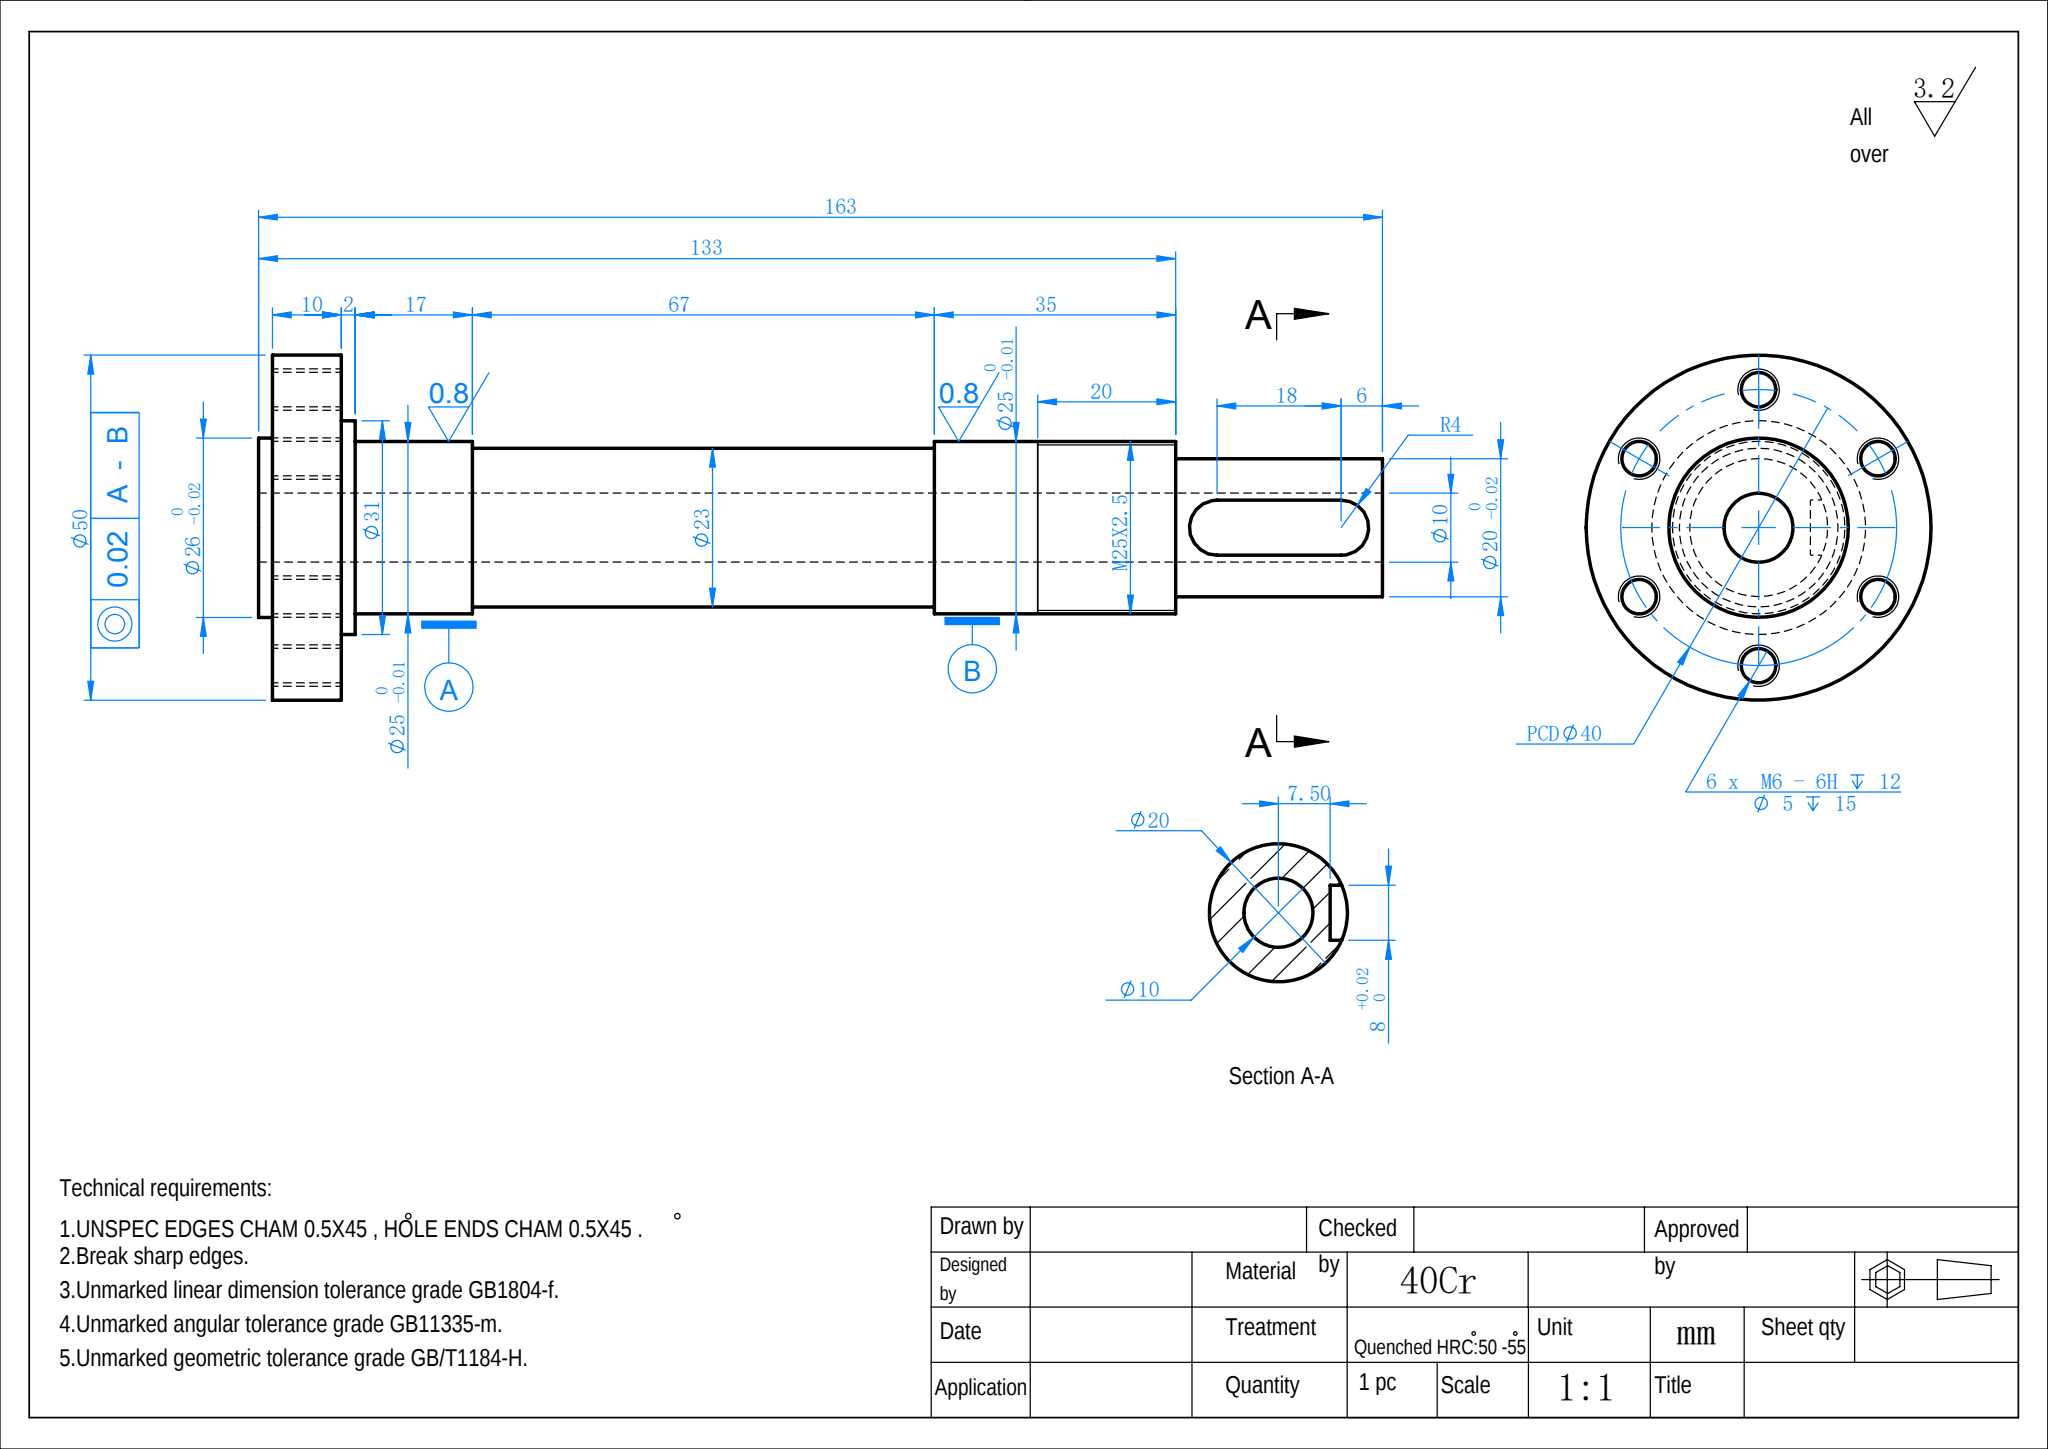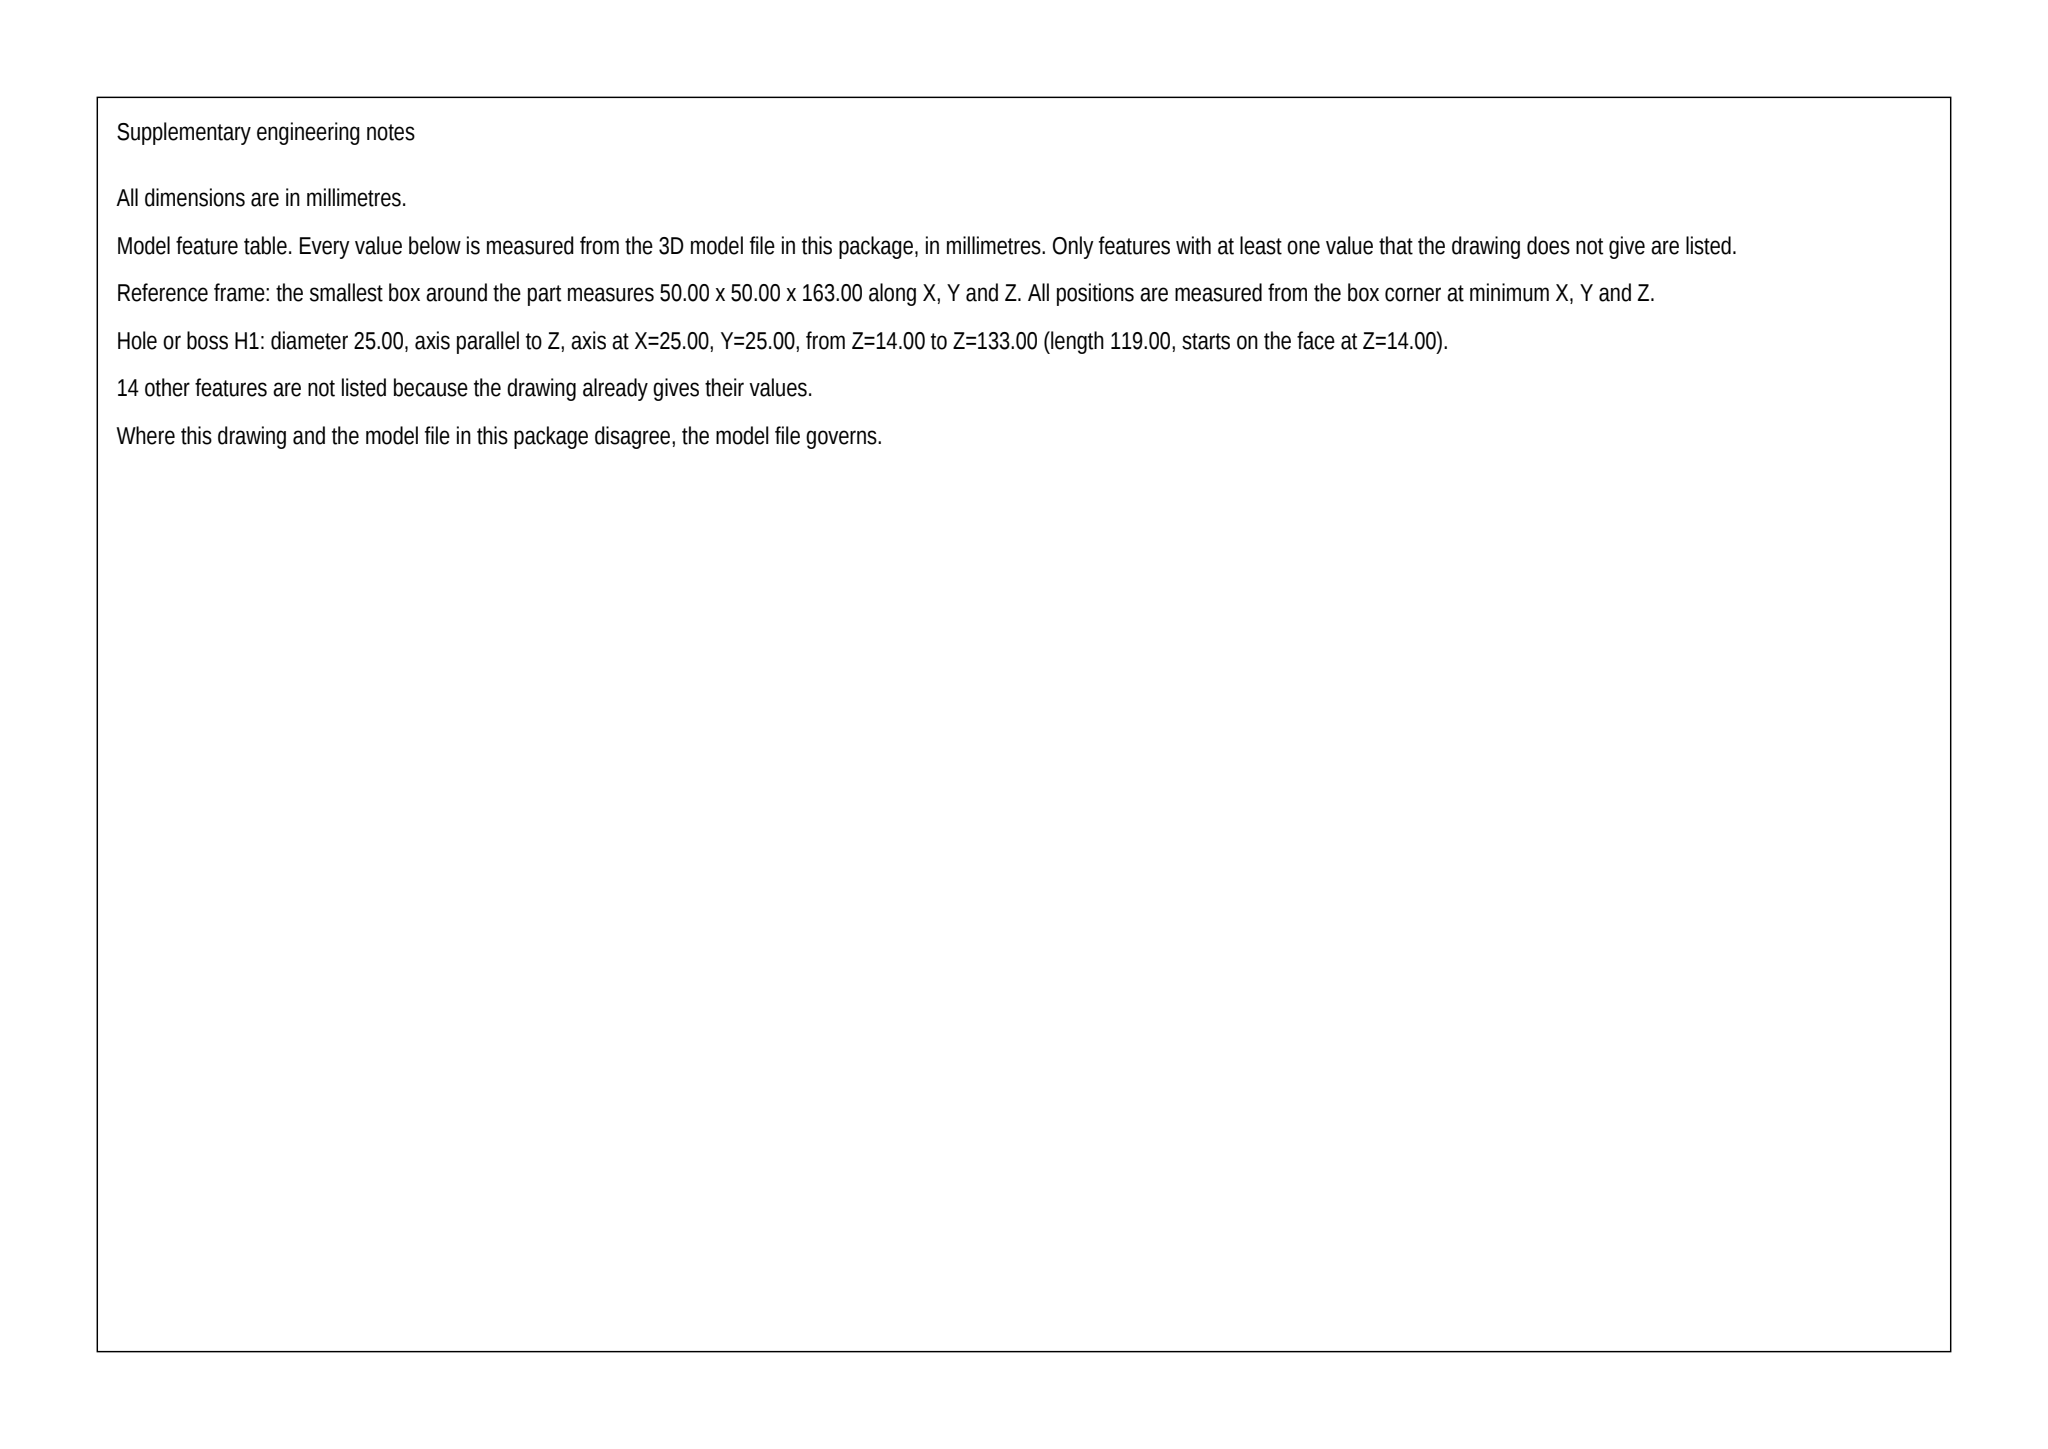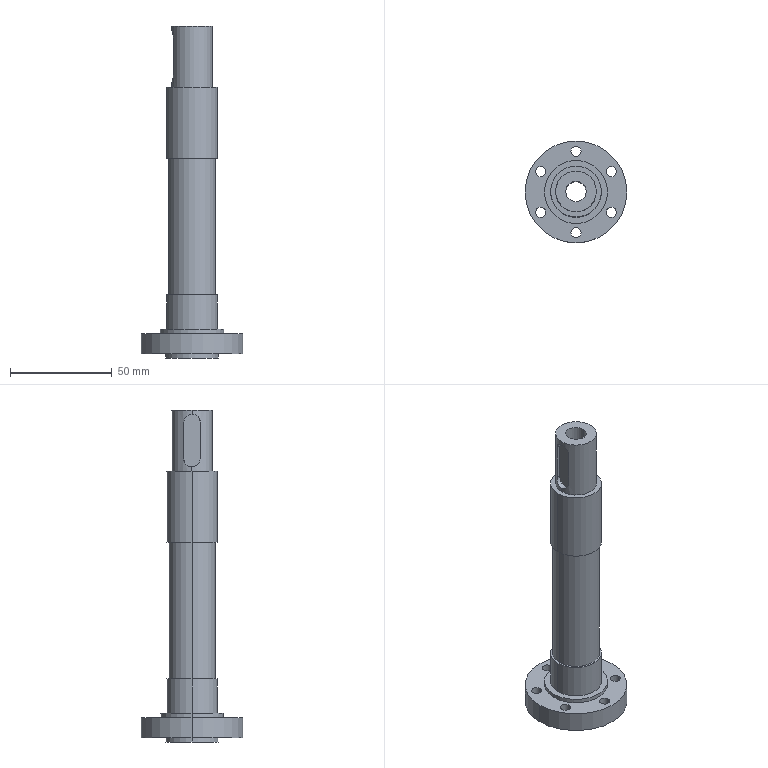Part | SolidWorks | mm | 1 solid | 42 faces | box 50 x 50 x 163 mm | volume 70577 mm3 | cylinder 31 | plane 11 | commonest cylinder face diameters 5 x12 25 x4 8 x3 10 x2 20 x2 23 x2 31 x2 26 x2
build123d program:
from build123d import *

# Parameters (mm, degrees)
SKETCH1_R           = 25
BOSS_EXTRUDE1_DEPTH = 10
SKETCH2_R           = 13
BOSS_EXTRUDE2_DEPTH = 2
SKETCH3_R           = 15.5
BOSS_EXTRUDE3_DEPTH = 2
SKETCH4_R           = 12.5
BOSS_EXTRUDE4_DEPTH = 17
SKETCH5_R           = 11.5
BOSS_EXTRUDE5_DEPTH = 67
SKETCH6_R           = 12.5
BOSS_EXTRUDE6_DEPTH = 35
SKETCH7_R           = 10
BOSS_EXTRUDE7_DEPTH = 30
CIRPATTERN1_COUNT   = 6
SKETCH11_R          = 5
CUT_EXTRUDE1_DEPTH  = 167.79
CUT_EXTRUDE2_DEPTH  = 2.5


with BuildPart() as part:
    # Sketch1 → Boss-Extrude1 (new body)
    with BuildSketch(Plane.XY):
        Circle(SKETCH1_R)
    extrude(amount=BOSS_EXTRUDE1_DEPTH)

    # Sketch2 → Boss-Extrude2 (add)
    with BuildSketch(Plane(origin=(0, 0, 0), x_dir=(-1, 0, 0), z_dir=(0, 0, -1))):
        with Locations(Location((0, 0, 0), (0, 0, 180))):
            Circle(SKETCH2_R)
    extrude(amount=BOSS_EXTRUDE2_DEPTH)

    # Sketch3 → Boss-Extrude3 (add)
    with BuildSketch(Plane.XY.offset(10)):
        Circle(SKETCH3_R)
    extrude(amount=BOSS_EXTRUDE3_DEPTH)

    # Sketch4 → Boss-Extrude4 (add)
    with BuildSketch(Plane.XY.offset(12)):
        Circle(SKETCH4_R)
    extrude(amount=BOSS_EXTRUDE4_DEPTH)

    # Sketch5 → Boss-Extrude5 (add)
    with BuildSketch(Plane.XY.offset(29)):
        Circle(SKETCH5_R)
    extrude(amount=BOSS_EXTRUDE5_DEPTH)

    # Sketch6 → Boss-Extrude6 (add)
    with BuildSketch(Plane.XY.offset(96)):
        Circle(SKETCH6_R)
    extrude(amount=BOSS_EXTRUDE6_DEPTH)

    # Sketch7 → Boss-Extrude7 (add)
    with BuildSketch(Plane.XY.offset(131)):
        Circle(SKETCH7_R)
    extrude(amount=BOSS_EXTRUDE7_DEPTH)

    # Sketch10 → M6 Tapped Hole1 (revolve, cut)
    with BuildSketch(Plane(origin=(0, 20, 0), x_dir=(0, 1, 0), z_dir=(1, 0, 0))):
        Polygon((0, 0), (0, 16.502), (2.5, 15), (2.5, 0), align=None)
    m6_tapped_hole1 = revolve(axis=Axis((0, 20, -6.35), (0, 0, 1)), mode=Mode.SUBTRACT)

    # CirPattern1: M6 Tapped Hole1 ×6 about axis
    cirpattern1_axis = Axis((0, 0, 0), (0, 0, 1))
    for i in range(1, CIRPATTERN1_COUNT):
        add(m6_tapped_hole1.rotate(cirpattern1_axis, i * 360 / CIRPATTERN1_COUNT), mode=Mode.SUBTRACT)

    # Sketch11 → Cut-Extrude1 (cut, through all)
    with BuildSketch(Plane.XY.offset(161)):
        Circle(SKETCH11_R)
    extrude(amount=-CUT_EXTRUDE1_DEPTH, mode=Mode.SUBTRACT)

    # Sketch12 → Cut-Extrude2 (cut)
    with BuildSketch(Plane.ZY.offset(10)):
        with BuildLine():
            Line((137, 4), (155, 4))
            ThreePointArc((155, 4), (159, 0), (155, -4))
            Line((155, -4), (137, -4))
            ThreePointArc((137, -4), (133, 0), (137, 4))
        make_face()
    extrude(amount=-CUT_EXTRUDE2_DEPTH, mode=Mode.SUBTRACT)


solid = part.part